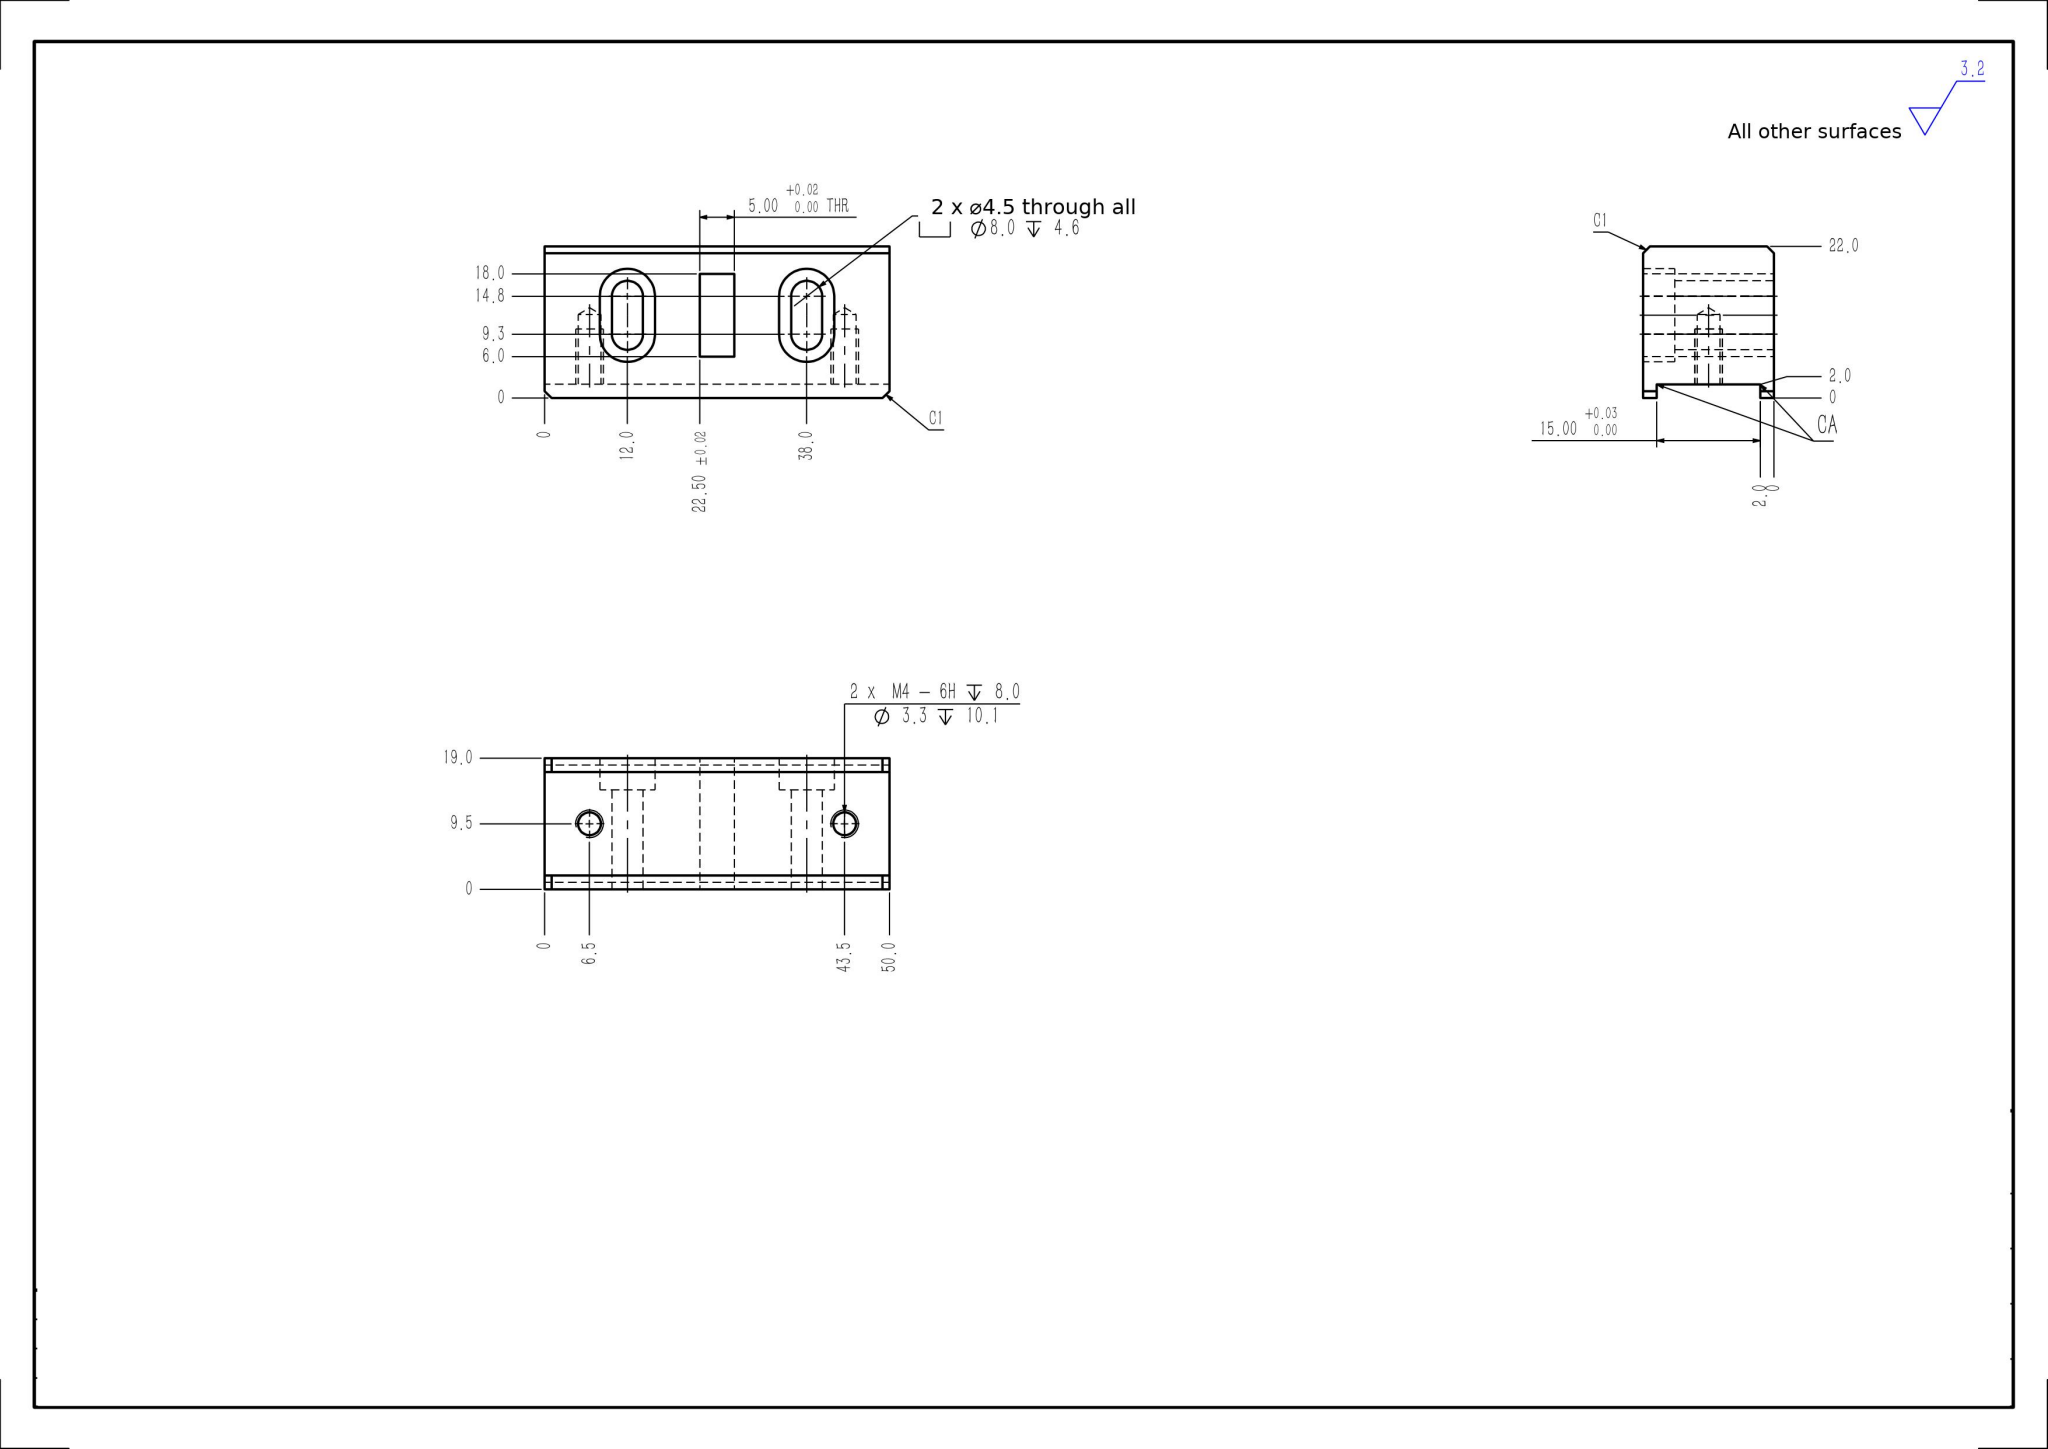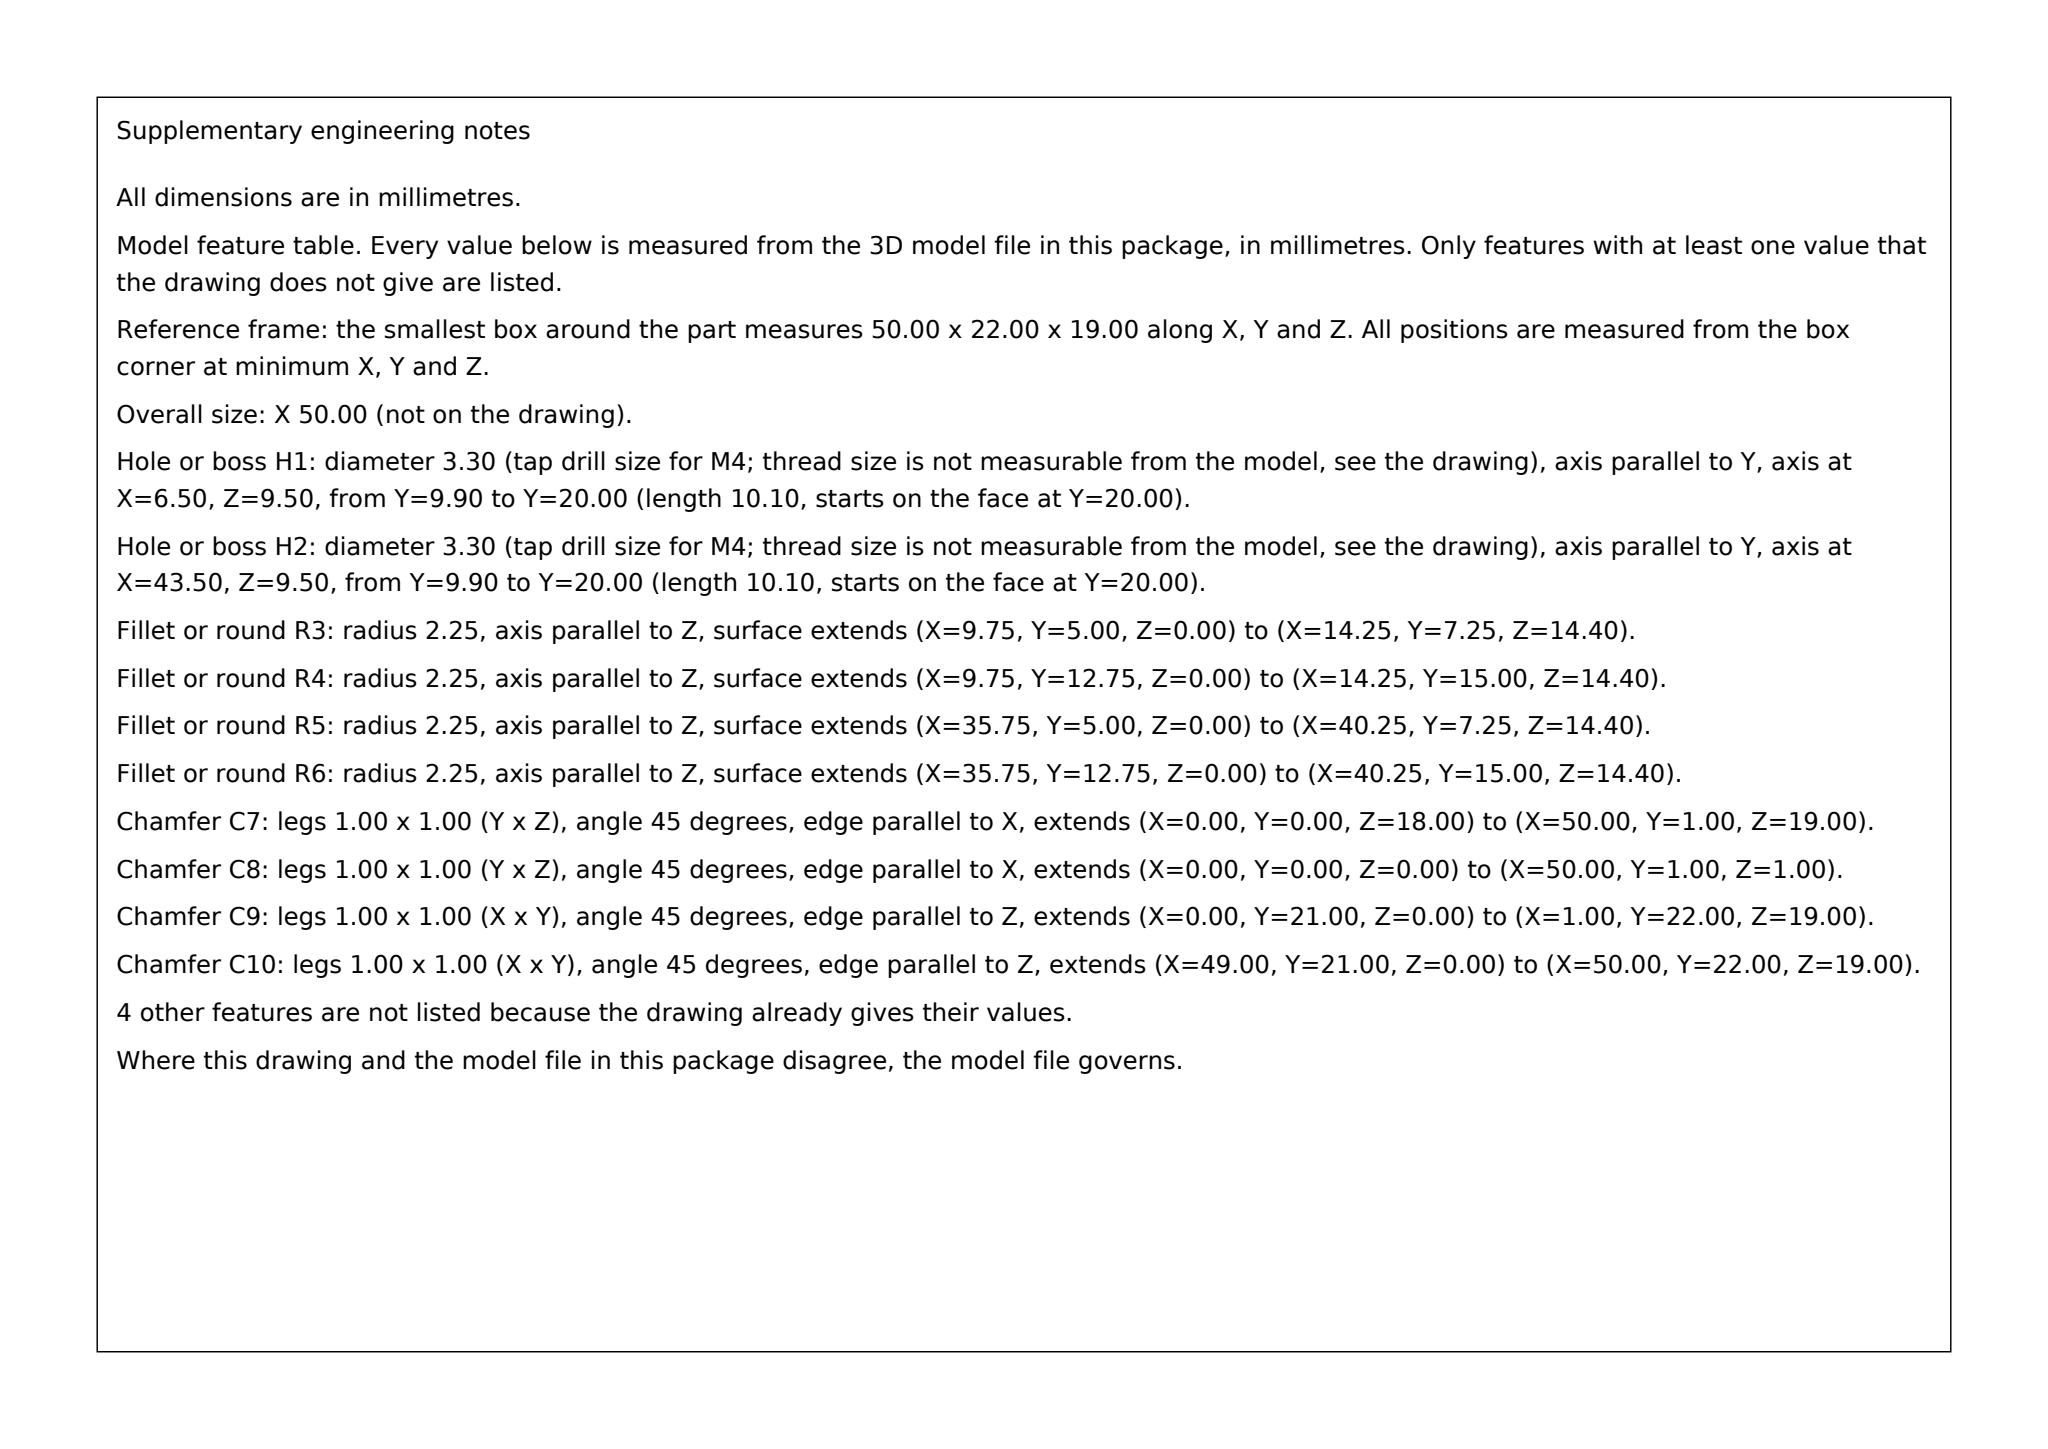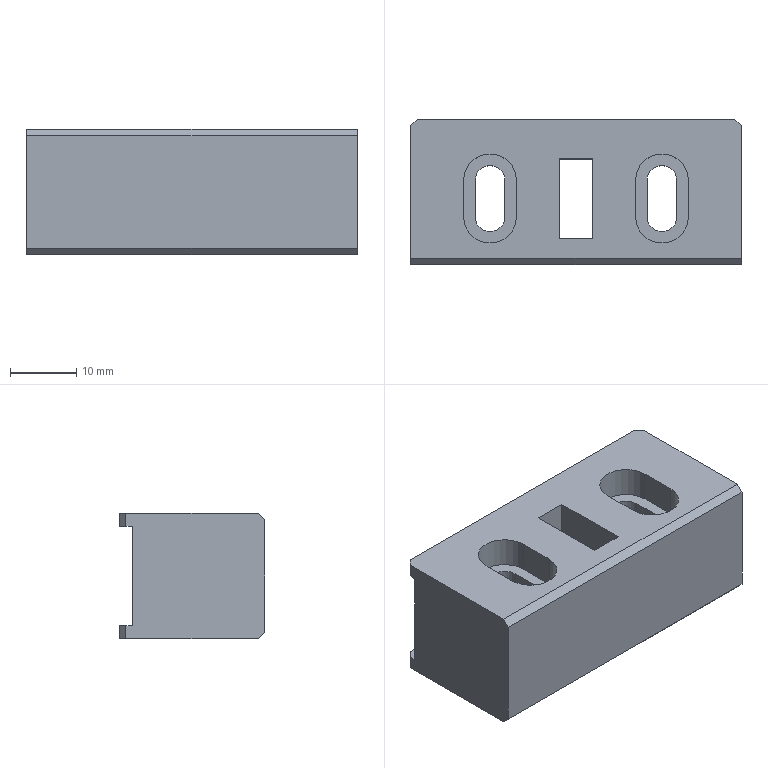Part | SolidWorks | mm | 1 solid | 46 faces | box 50 x 22 x 19 mm | volume 15989 mm3 | plane 30 | cylinder 12 | cone 4 | commonest cylinder face diameters 3.3 x4 4.5 x4 8 x4